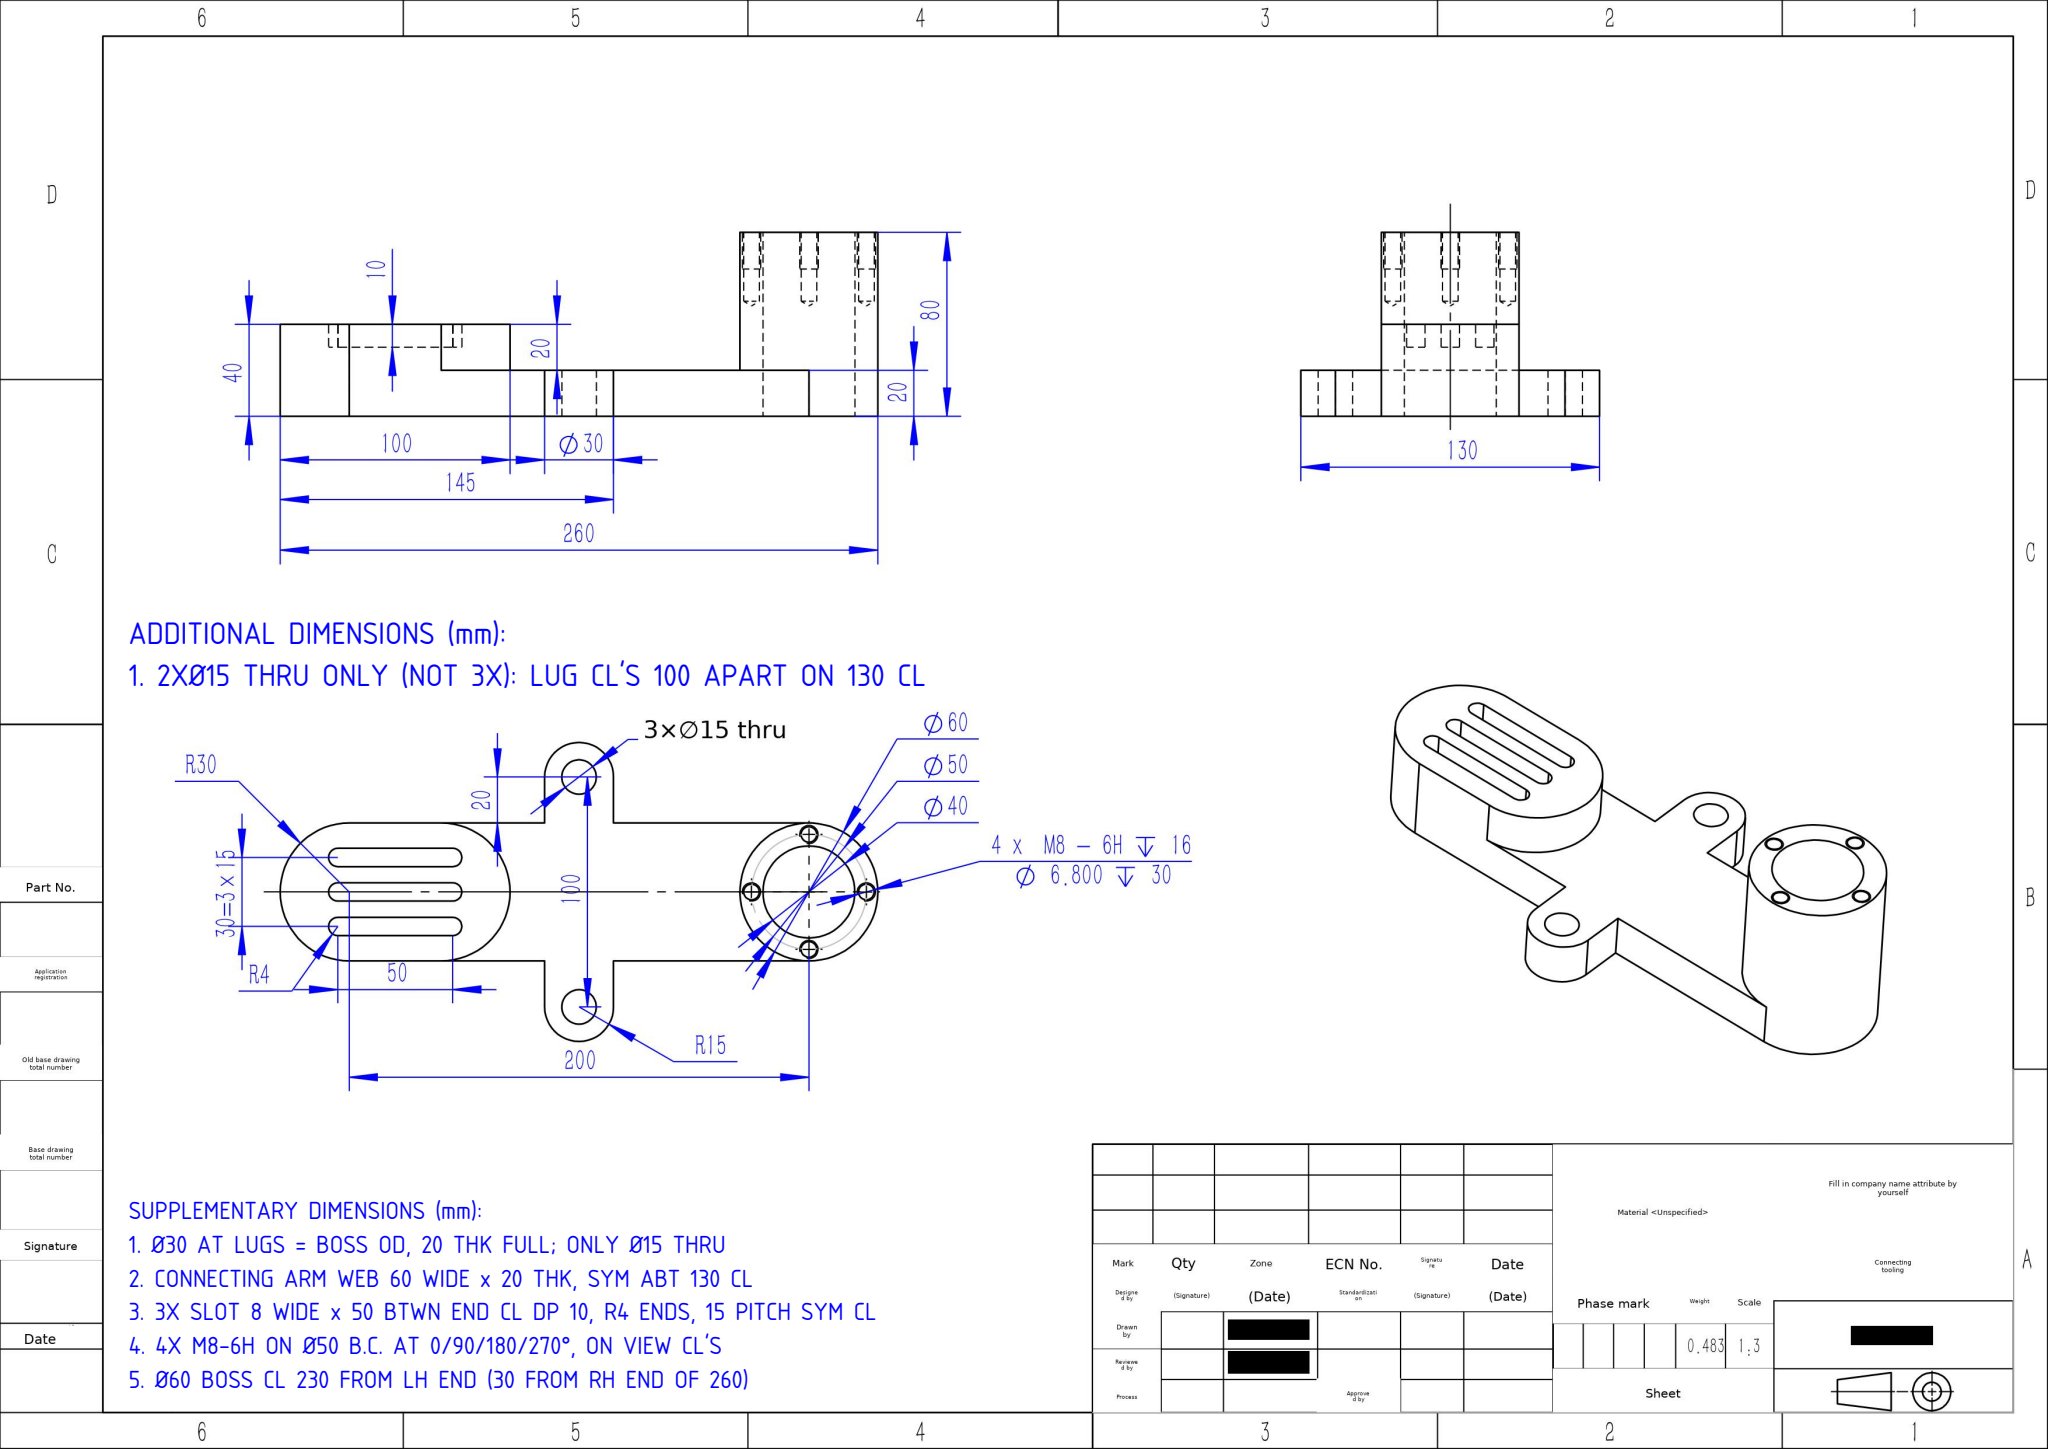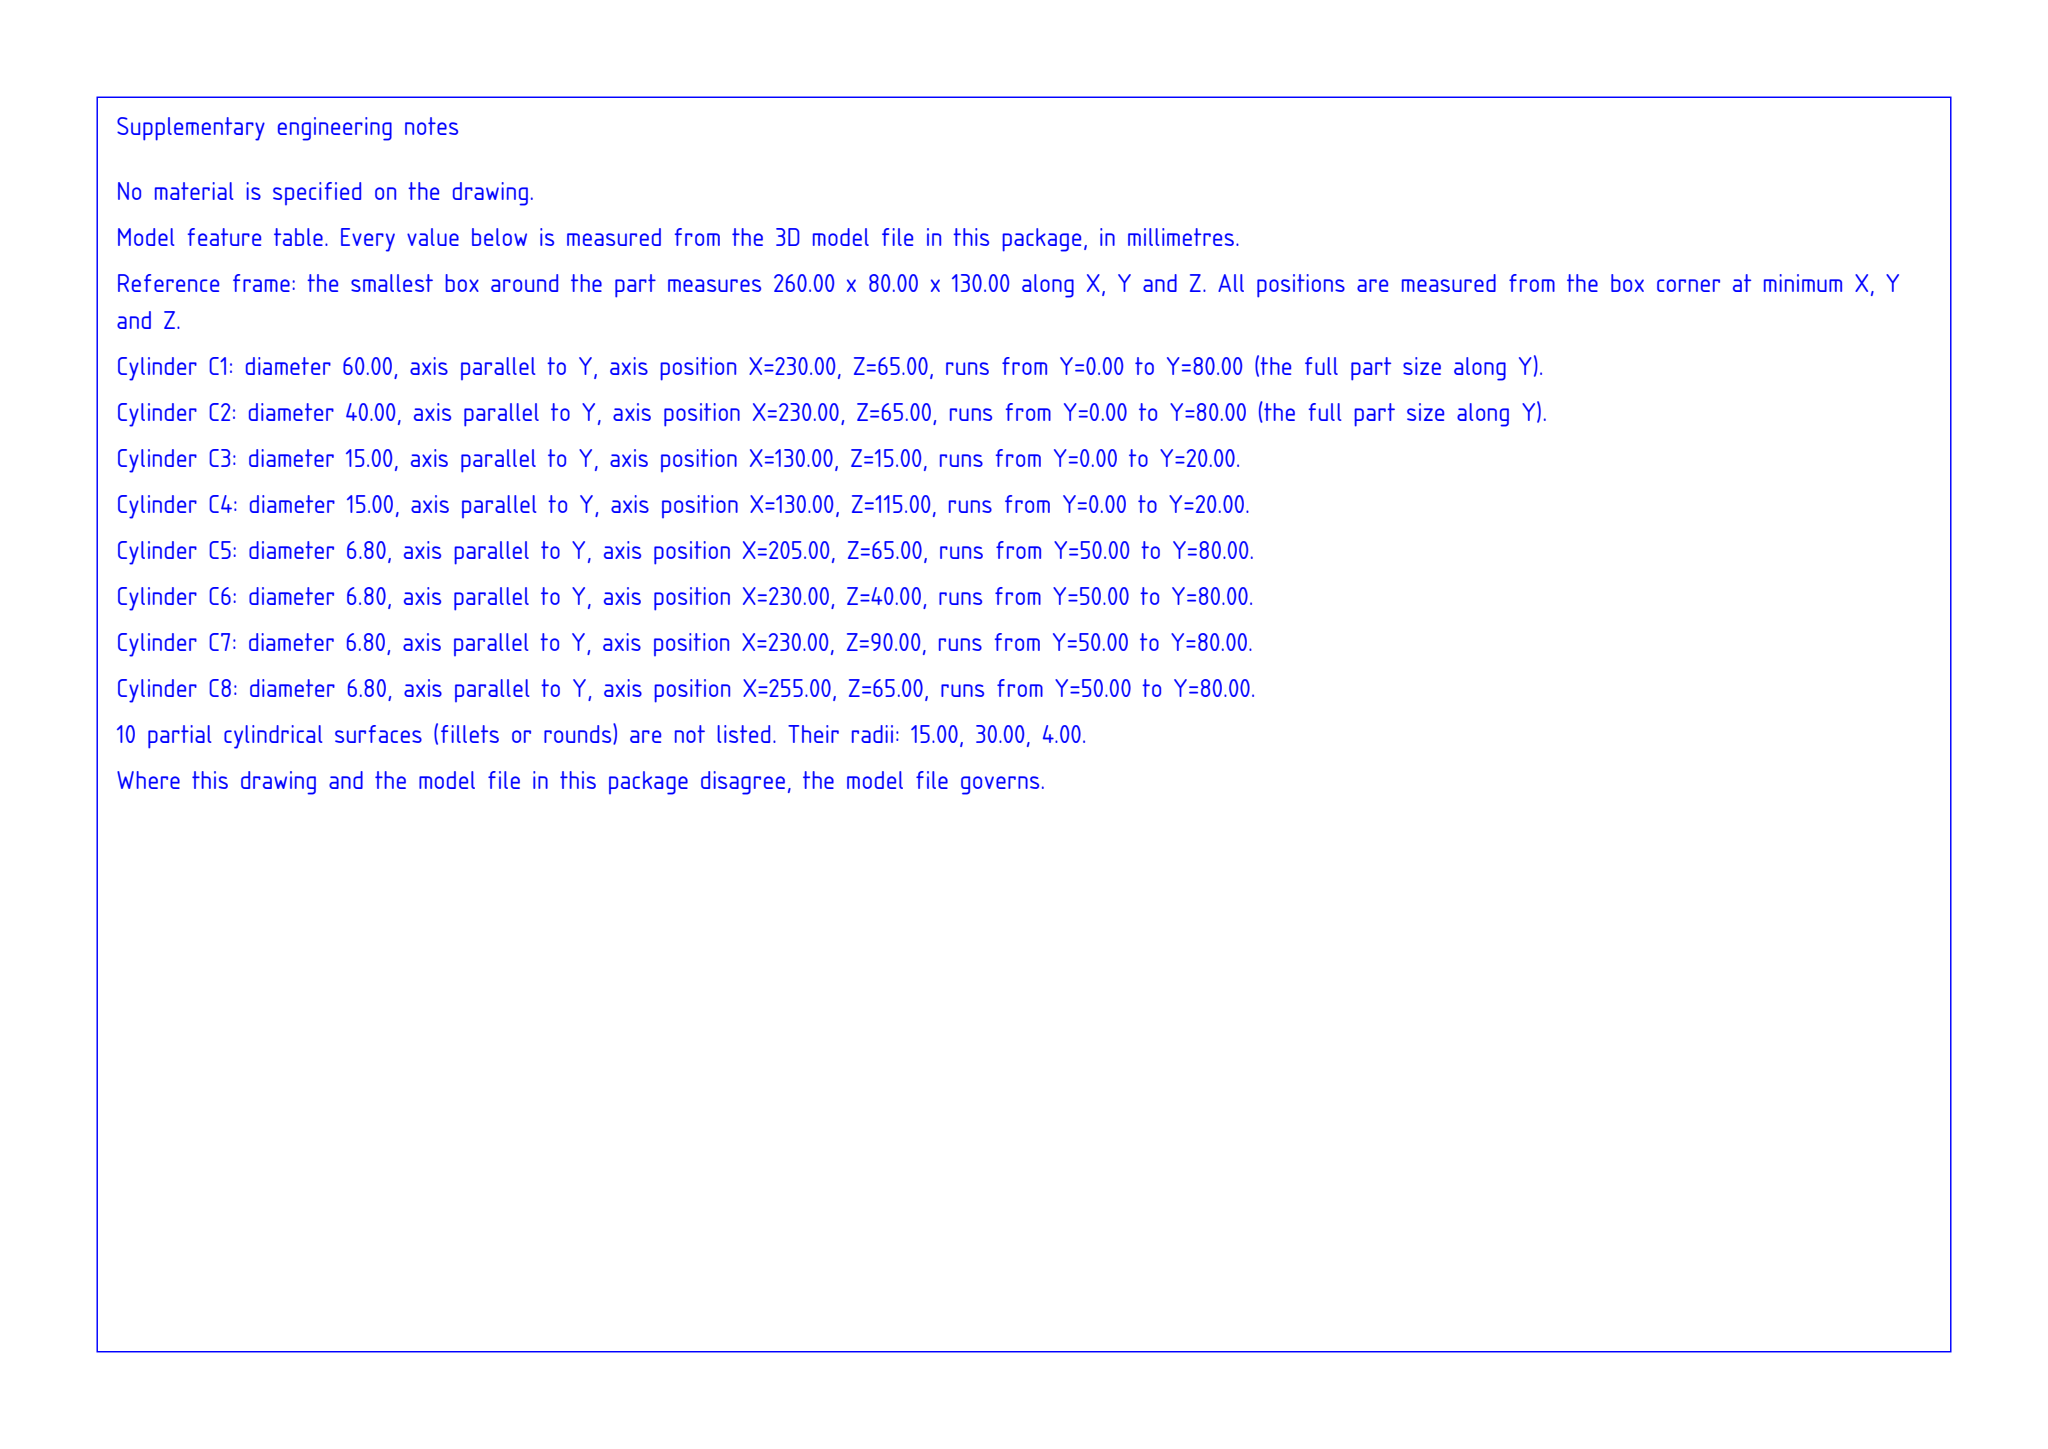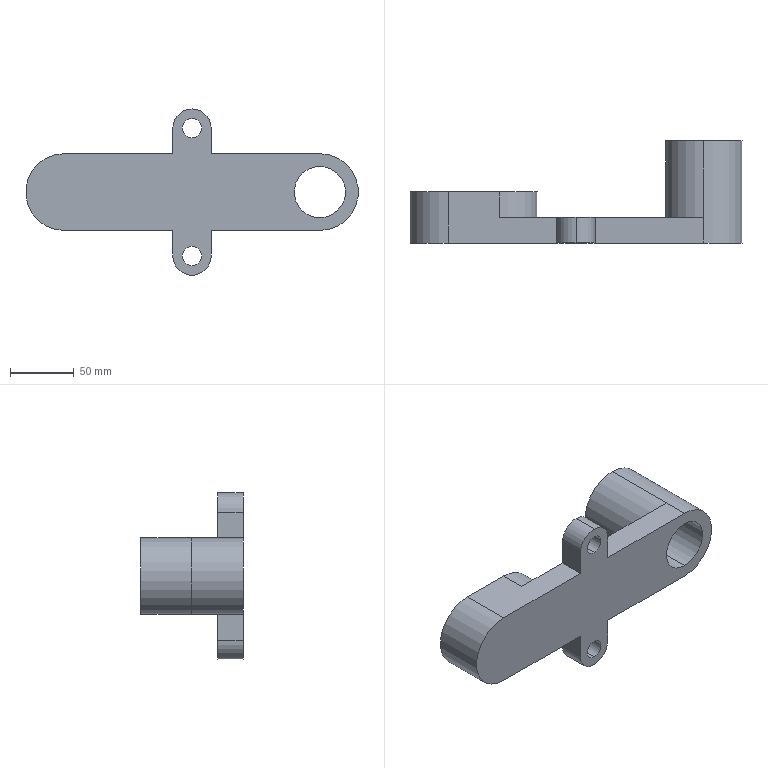Part | SolidWorks | mm | 1 solid | 56 faces | box 260 x 80 x 130 mm | volume 483316 mm3 | cylinder 27 | plane 21 | cone 8 | commonest cylinder face diameters 6.8 x8 8 x6 15 x4 60 x4 30 x3 40 x2